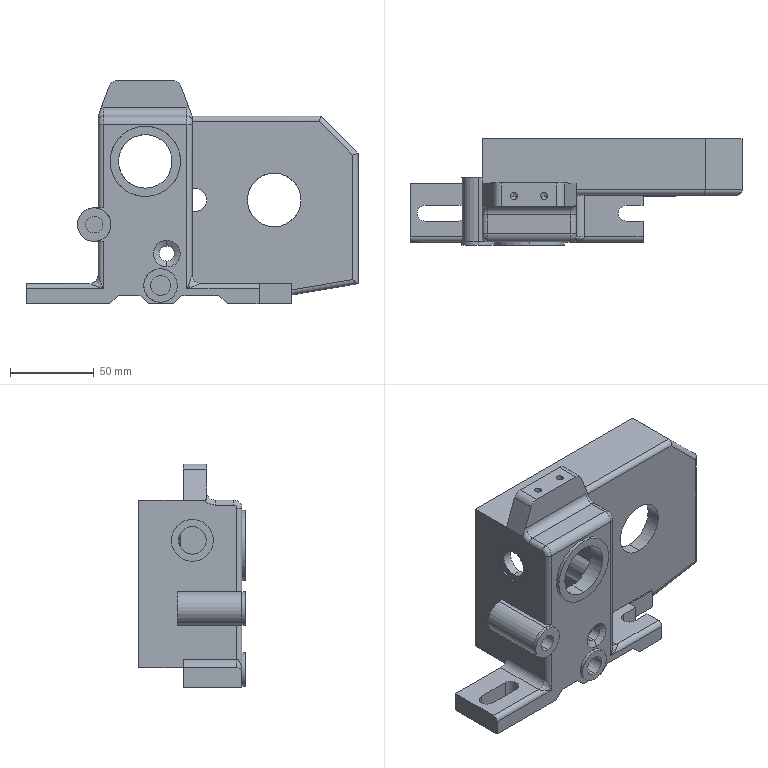CAM job | Mastercam | mm | 5 operations | part box 198 x 63.5 x 133.5
1. Drill/Counterbore | 12 - 12 定位钻
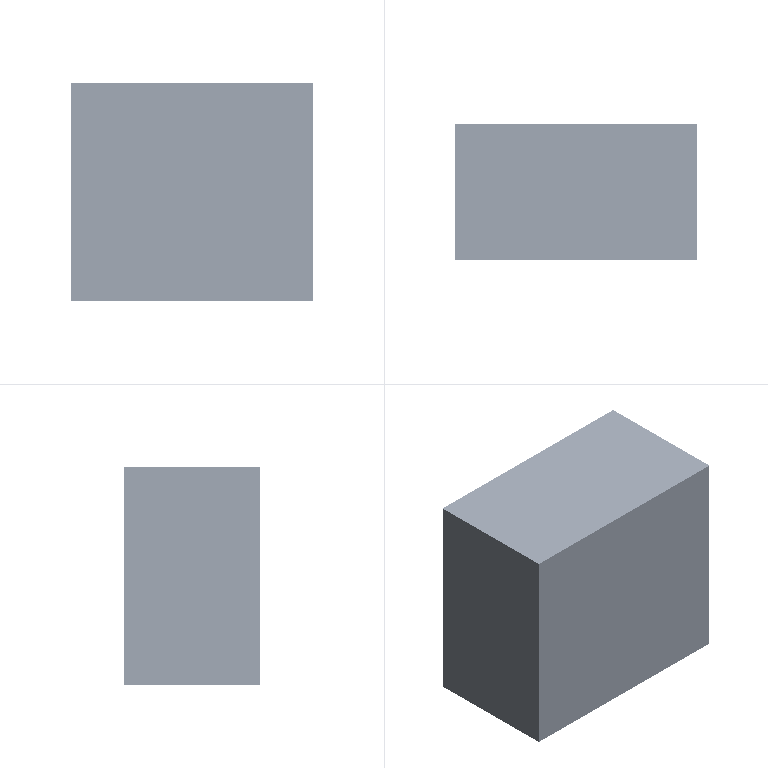2. Drill/Counterbore | 12 - 12 定位钻
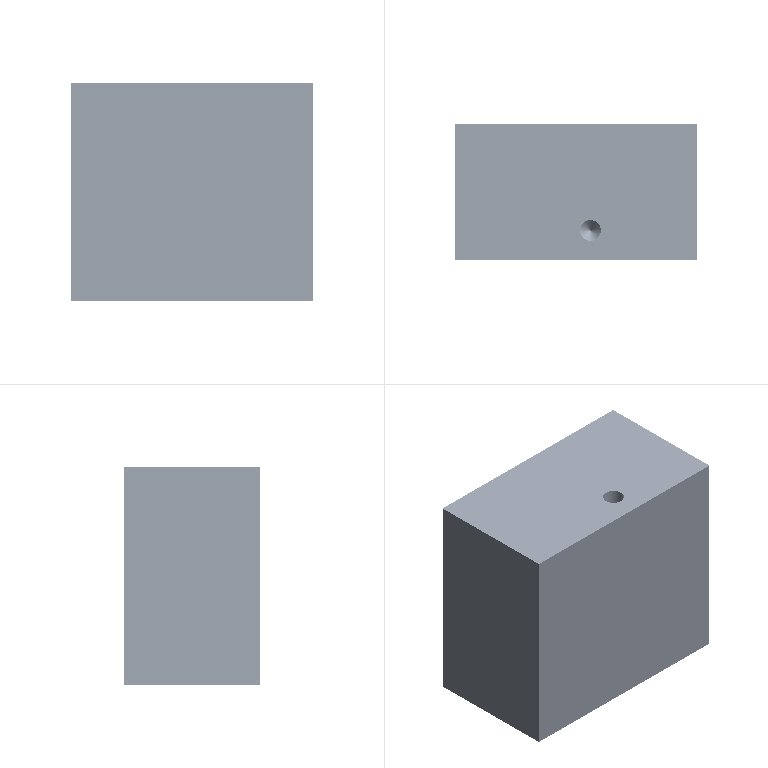3. Peck Drill | 1 - 4.3 钻头
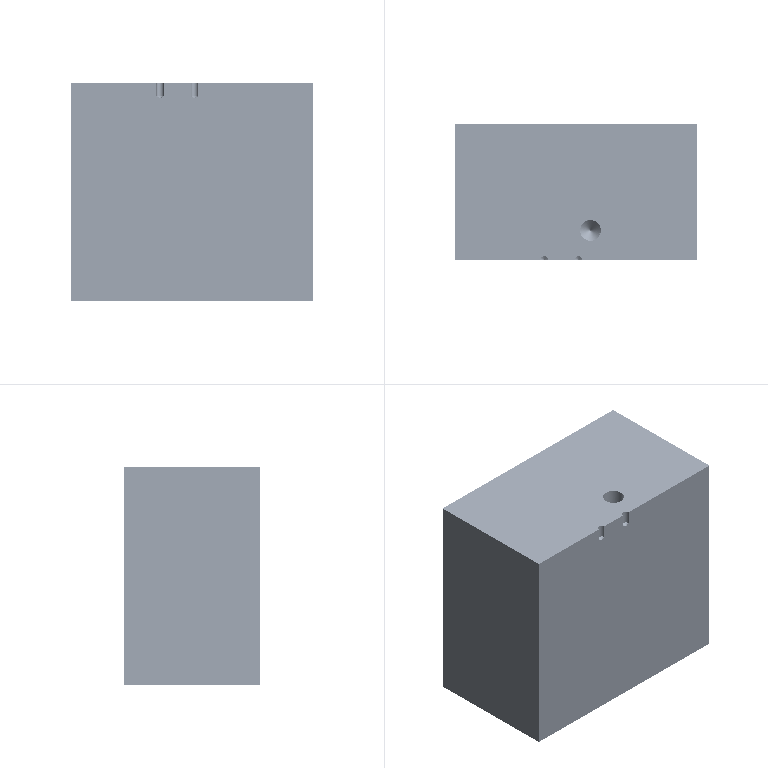4. Peck Drill | 24 - 9 钻头
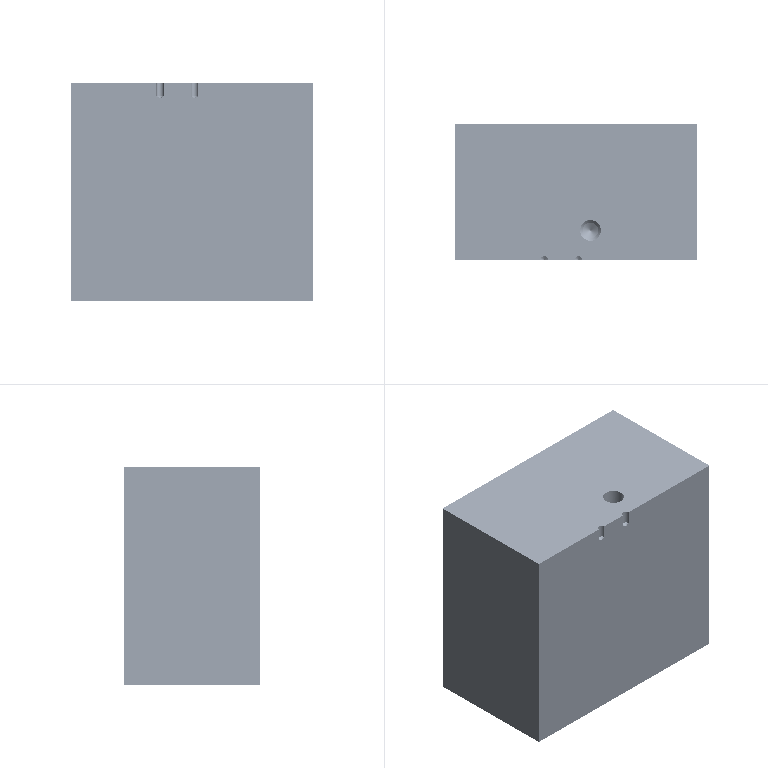5. Contour (Ramp) | 22 - 8 平铣刀